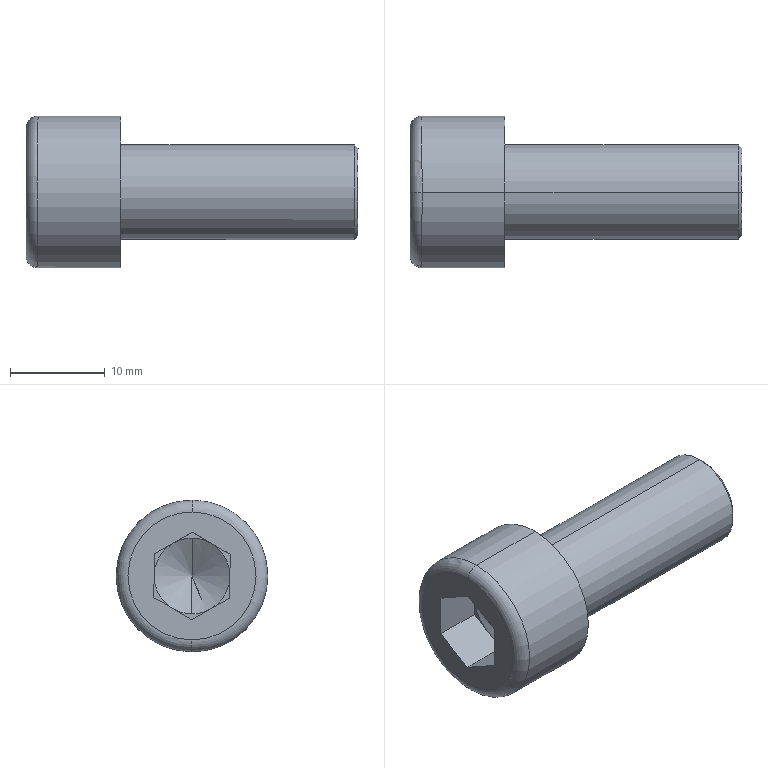Component | SolidWorks | hexagon socket head cap screws gb-29 | 1 solid | 25 faces | box 35.01 x 16 x 16.01 mm | volume 3640 mm3 | plane 15 | cone 4 | cylinder 4 | torus 2 | commonest cylinder face diameters 10 x2 16 x2
STEP:
#1=CARTESIAN_POINT('',(-1.117,35.713,19.655));
#2=VERTEX_POINT('',#1);
#3=CARTESIAN_POINT('',(-1.117,35.71,20.017));
#4=VERTEX_POINT('',#3);
#5=CARTESIAN_POINT('',(-1.117,35.712,19.836));
#6=DIRECTION('',(1.,0.,-0.00108));
#7=DIRECTION('',(-0.00108,0.008644,-1.));
#8=AXIS2_PLACEMENT_3D('',#5,#6,#7);
#9=CIRCLE('',#8,0.1811);
#10=EDGE_CURVE('',#2,#4,#9,.T.);
#11=ORIENTED_EDGE('',*,*,#10,.F.);
#12=CARTESIAN_POINT('',(-1.133,35.714,19.639));
#13=VERTEX_POINT('',#12);
#14=CARTESIAN_POINT('',(-1.117,35.713,19.655));
#15=DIRECTION('',(-0.7079,0.006112,-0.7063));
#16=VECTOR('',#15,39.37);
#17=LINE('',#14,#16);
#18=EDGE_CURVE('',#2,#13,#17,.T.);
#19=ORIENTED_EDGE('',*,*,#18,.T.);
#20=CARTESIAN_POINT('',(-1.133,35.71,20.033));
#21=VERTEX_POINT('',#20);
#22=CARTESIAN_POINT('',(-1.133,35.712,19.836));
#23=DIRECTION('',(-1.,-0.,0.00108));
#24=DIRECTION('',(-0.00108,0.008644,-1.));
#25=AXIS2_PLACEMENT_3D('',#22,#23,#24);
#26=CIRCLE('',#25,0.1969);
#27=EDGE_CURVE('',#21,#13,#26,.T.);
#28=ORIENTED_EDGE('',*,*,#27,.F.);
#29=CARTESIAN_POINT('',(-1.117,35.71,20.017));
#30=DIRECTION('',(-0.7063,-0.006112,0.7078));
#31=VECTOR('',#30,39.37);
#32=LINE('',#29,#31);
#33=EDGE_CURVE('',#4,#21,#32,.T.);
#34=ORIENTED_EDGE('',*,*,#33,.F.);
#35=EDGE_LOOP('',(#11,#19,#28,#34));
#36=FACE_OUTER_BOUND('',#35,.T.);
#37=CARTESIAN_POINT('',(-1.117,35.712,19.836));
#38=DIRECTION('',(-1.,-0.,0.00108));
#39=DIRECTION('',(0.00108,-0.008644,1.));
#40=AXIS2_PLACEMENT_3D('',#37,#38,#39);
#41=CONICAL_SURFACE('',#40,0.1811,0.7854);
#42=ADVANCED_FACE('',(#36),#41,.T.);
#43=CARTESIAN_POINT('',(-2.495,35.71,20.103));
#44=VERTEX_POINT('',#43);
#45=CARTESIAN_POINT('',(-2.495,35.714,19.572));
#46=VERTEX_POINT('',#45);
#47=CARTESIAN_POINT('',(-2.495,35.712,19.837));
#48=DIRECTION('',(-1.,-0.,0.00108));
#49=DIRECTION('',(-0.00108,0.008644,-1.));
#50=AXIS2_PLACEMENT_3D('',#47,#48,#49);
#51=CIRCLE('',#50,0.2657);
#52=EDGE_CURVE('',#44,#46,#51,.T.);
#53=ORIENTED_EDGE('',*,*,#52,.F.);
#54=CARTESIAN_POINT('',(-2.446,35.709,20.152));
#55=VERTEX_POINT('',#54);
#56=CARTESIAN_POINT('',(-2.446,35.71,20.103));
#57=DIRECTION('',(0.00000934,1.,0.008644));
#58=DIRECTION('',(0.,-0.008644,1.));
#59=AXIS2_PLACEMENT_3D('',#56,#57,#58);
#60=CIRCLE('',#59,0.04921);
#61=EDGE_CURVE('',#44,#55,#60,.T.);
#62=ORIENTED_EDGE('',*,*,#61,.T.);
#63=CARTESIAN_POINT('',(-2.446,35.715,19.522));
#64=VERTEX_POINT('',#63);
#65=CARTESIAN_POINT('',(-2.446,35.712,19.837));
#66=DIRECTION('',(1.,0.,-0.00108));
#67=DIRECTION('',(-0.00108,0.008644,-1.));
#68=AXIS2_PLACEMENT_3D('',#65,#66,#67);
#69=CIRCLE('',#68,0.315);
#70=EDGE_CURVE('',#64,#55,#69,.T.);
#71=ORIENTED_EDGE('',*,*,#70,.F.);
#72=CARTESIAN_POINT('',(-2.446,35.714,19.571));
#73=DIRECTION('',(-0.00000934,-1.,-0.008644));
#74=DIRECTION('',(0.,0.008644,-1.));
#75=AXIS2_PLACEMENT_3D('',#72,#73,#74);
#76=CIRCLE('',#75,0.04921);
#77=EDGE_CURVE('',#46,#64,#76,.T.);
#78=ORIENTED_EDGE('',*,*,#77,.F.);
#79=EDGE_LOOP('',(#53,#62,#71,#78));
#80=FACE_OUTER_BOUND('',#79,.T.);
#81=CARTESIAN_POINT('',(-2.446,35.712,19.837));
#82=DIRECTION('',(1.,0.,-0.00108));
#83=DIRECTION('',(-0.00108,0.008644,-1.));
#84=AXIS2_PLACEMENT_3D('',#81,#82,#83);
#85=TOROIDAL_SURFACE('',#84,0.2657,0.04921);
#86=ADVANCED_FACE('',(#80),#85,.T.);
#87=CARTESIAN_POINT('',(-2.207,35.712,19.837));
#88=VERTEX_POINT('',#87);
#89=CARTESIAN_POINT('',(-2.298,35.711,19.994));
#90=VERTEX_POINT('',#89);
#91=CARTESIAN_POINT('',(-2.298,35.711,19.994));
#92=DIRECTION('',(-0.4991,-0.007486,0.8665));
#93=VECTOR('',#92,39.37);
#94=LINE('',#91,#93);
#95=EDGE_CURVE('',#88,#90,#94,.T.);
#96=ORIENTED_EDGE('',*,*,#95,.F.);
#97=CARTESIAN_POINT('',(-2.298,35.713,19.68));
#98=VERTEX_POINT('',#97);
#99=CARTESIAN_POINT('',(-2.298,35.713,19.68));
#100=DIRECTION('',(-0.5009,0.007486,-0.8655));
#101=VECTOR('',#100,39.37);
#102=LINE('',#99,#101);
#103=EDGE_CURVE('',#88,#98,#102,.T.);
#104=ORIENTED_EDGE('',*,*,#103,.T.);
#105=CARTESIAN_POINT('',(-2.298,35.634,19.7));
#106=VERTEX_POINT('',#105);
#107=CARTESIAN_POINT('',(-2.298,35.712,19.837));
#108=DIRECTION('',(1.,0.,-0.00108));
#109=DIRECTION('',(0.00108,-0.008644,1.));
#110=AXIS2_PLACEMENT_3D('',#107,#108,#109);
#111=CIRCLE('',#110,0.1575);
#112=EDGE_CURVE('',#106,#98,#111,.T.);
#113=ORIENTED_EDGE('',*,*,#112,.F.);
#114=CARTESIAN_POINT('',(-2.298,35.554,19.836));
#115=VERTEX_POINT('',#114);
#116=CARTESIAN_POINT('',(-2.298,35.712,19.837));
#117=DIRECTION('',(1.,0.,-0.00108));
#118=DIRECTION('',(0.00108,-0.008644,1.));
#119=AXIS2_PLACEMENT_3D('',#116,#117,#118);
#120=CIRCLE('',#119,0.1575);
#121=EDGE_CURVE('',#115,#106,#120,.T.);
#122=ORIENTED_EDGE('',*,*,#121,.F.);
#123=CARTESIAN_POINT('',(-2.298,35.632,19.973));
#124=VERTEX_POINT('',#123);
#125=CARTESIAN_POINT('',(-2.298,35.712,19.837));
#126=DIRECTION('',(1.,0.,-0.00108));
#127=DIRECTION('',(0.00108,-0.008644,1.));
#128=AXIS2_PLACEMENT_3D('',#125,#126,#127);
#129=CIRCLE('',#128,0.1575);
#130=EDGE_CURVE('',#124,#115,#129,.T.);
#131=ORIENTED_EDGE('',*,*,#130,.F.);
#132=CARTESIAN_POINT('',(-2.298,35.712,19.837));
#133=DIRECTION('',(1.,0.,-0.00108));
#134=DIRECTION('',(0.00108,-0.008644,1.));
#135=AXIS2_PLACEMENT_3D('',#132,#133,#134);
#136=CIRCLE('',#135,0.1575);
#137=EDGE_CURVE('',#90,#124,#136,.T.);
#138=ORIENTED_EDGE('',*,*,#137,.F.);
#139=EDGE_LOOP('',(#96,#104,#113,#122,#131,#138));
#140=FACE_OUTER_BOUND('',#139,.T.);
#141=CARTESIAN_POINT('',(-2.298,35.712,19.837));
#142=DIRECTION('',(-1.,-0.,0.00108));
#143=DIRECTION('',(0.00108,-0.008644,1.));
#144=AXIS2_PLACEMENT_3D('',#141,#142,#143);
#145=CONICAL_SURFACE('',#144,0.1575,1.047);
#146=ADVANCED_FACE('',(#140),#145,.F.);
#147=ORIENTED_EDGE('',*,*,#27,.T.);
#148=CARTESIAN_POINT('',(-2.102,35.714,19.64));
#149=VERTEX_POINT('',#148);
#150=CARTESIAN_POINT('',(-1.117,35.714,19.639));
#151=DIRECTION('',(-1.,-0.,0.00108));
#152=VECTOR('',#151,39.37);
#153=LINE('',#150,#152);
#154=EDGE_CURVE('',#13,#149,#153,.T.);
#155=ORIENTED_EDGE('',*,*,#154,.T.);
#156=CARTESIAN_POINT('',(-2.101,35.71,20.034));
#157=VERTEX_POINT('',#156);
#158=CARTESIAN_POINT('',(-2.101,35.712,19.837));
#159=DIRECTION('',(1.,0.,-0.00108));
#160=DIRECTION('',(-0.00108,0.008644,-1.));
#161=AXIS2_PLACEMENT_3D('',#158,#159,#160);
#162=CIRCLE('',#161,0.1969);
#163=EDGE_CURVE('',#149,#157,#162,.T.);
#164=ORIENTED_EDGE('',*,*,#163,.T.);
#165=CARTESIAN_POINT('',(-1.117,35.71,20.033));
#166=DIRECTION('',(-1.,-0.,0.00108));
#167=VECTOR('',#166,39.37);
#168=LINE('',#165,#167);
#169=EDGE_CURVE('',#21,#157,#168,.T.);
#170=ORIENTED_EDGE('',*,*,#169,.F.);
#171=EDGE_LOOP('',(#147,#155,#164,#170));
#172=FACE_OUTER_BOUND('',#171,.T.);
#173=CARTESIAN_POINT('',(-1.117,35.712,19.836));
#174=DIRECTION('',(-1.,-0.,0.00108));
#175=DIRECTION('',(0.00108,-0.008644,1.));
#176=AXIS2_PLACEMENT_3D('',#173,#174,#175);
#177=CYLINDRICAL_SURFACE('',#176,0.1969);
#178=ADVANCED_FACE('',(#172),#177,.T.);
#179=CARTESIAN_POINT('',(-2.102,35.715,19.522));
#180=VERTEX_POINT('',#179);
#181=CARTESIAN_POINT('',(-2.101,35.709,20.152));
#182=VERTEX_POINT('',#181);
#183=CARTESIAN_POINT('',(-2.101,35.712,19.837));
#184=DIRECTION('',(1.,0.,-0.00108));
#185=DIRECTION('',(-0.00108,0.008644,-1.));
#186=AXIS2_PLACEMENT_3D('',#183,#184,#185);
#187=CIRCLE('',#186,0.315);
#188=EDGE_CURVE('',#180,#182,#187,.T.);
#189=ORIENTED_EDGE('',*,*,#188,.F.);
#190=CARTESIAN_POINT('',(-2.102,35.715,19.522));
#191=DIRECTION('',(-1.,-0.,0.00108));
#192=VECTOR('',#191,39.37);
#193=LINE('',#190,#192);
#194=EDGE_CURVE('',#180,#64,#193,.T.);
#195=ORIENTED_EDGE('',*,*,#194,.T.);
#196=ORIENTED_EDGE('',*,*,#70,.T.);
#197=CARTESIAN_POINT('',(-2.101,35.709,20.152));
#198=DIRECTION('',(-1.,-0.,0.00108));
#199=VECTOR('',#198,39.37);
#200=LINE('',#197,#199);
#201=EDGE_CURVE('',#182,#55,#200,.T.);
#202=ORIENTED_EDGE('',*,*,#201,.F.);
#203=EDGE_LOOP('',(#189,#195,#196,#202));
#204=FACE_OUTER_BOUND('',#203,.T.);
#205=CARTESIAN_POINT('',(-2.101,35.712,19.837));
#206=DIRECTION('',(-1.,-0.,0.00108));
#207=DIRECTION('',(0.00108,-0.008644,1.));
#208=AXIS2_PLACEMENT_3D('',#205,#206,#207);
#209=CYLINDRICAL_SURFACE('',#208,0.315);
#210=ADVANCED_FACE('',(#204),#209,.T.);
#211=CARTESIAN_POINT('',(-2.298,35.554,19.927));
#212=VERTEX_POINT('',#211);
#213=CARTESIAN_POINT('',(-2.298,35.71,20.019));
#214=DIRECTION('',(-0.0005483,-0.8617,-0.5075));
#215=VECTOR('',#214,39.37);
#216=LINE('',#213,#215);
#217=EDGE_CURVE('',#124,#212,#216,.T.);
#218=ORIENTED_EDGE('',*,*,#217,.F.);
#219=ORIENTED_EDGE('',*,*,#130,.T.);
#220=CARTESIAN_POINT('',(-2.298,35.554,19.927));
#221=DIRECTION('',(-0.00108,0.008644,-1.));
#222=VECTOR('',#221,39.37);
#223=LINE('',#220,#222);
#224=EDGE_CURVE('',#212,#115,#223,.T.);
#225=ORIENTED_EDGE('',*,*,#224,.F.);
#226=EDGE_LOOP('',(#218,#219,#225));
#227=FACE_OUTER_BOUND('',#226,.T.);
#228=CARTESIAN_POINT('',(-2.298,35.397,19.834));
#229=DIRECTION('',(-1.,-0.,0.00108));
#230=DIRECTION('',(0.00108,-0.008644,1.));
#231=AXIS2_PLACEMENT_3D('',#228,#229,#230);
#232=PLANE('',#231);
#233=ADVANCED_FACE('',(#227),#232,.T.);
#234=CARTESIAN_POINT('',(-2.298,35.555,19.745));
#235=VERTEX_POINT('',#234);
#236=CARTESIAN_POINT('',(-2.298,35.554,19.927));
#237=DIRECTION('',(-0.00108,0.008644,-1.));
#238=VECTOR('',#237,39.37);
#239=LINE('',#236,#238);
#240=EDGE_CURVE('',#115,#235,#239,.T.);
#241=ORIENTED_EDGE('',*,*,#240,.F.);
#242=ORIENTED_EDGE('',*,*,#121,.T.);
#243=CARTESIAN_POINT('',(-2.298,35.555,19.745));
#244=DIRECTION('',(-0.0005321,0.8703,-0.4925));
#245=VECTOR('',#244,39.37);
#246=LINE('',#243,#245);
#247=EDGE_CURVE('',#235,#106,#246,.T.);
#248=ORIENTED_EDGE('',*,*,#247,.F.);
#249=EDGE_LOOP('',(#241,#242,#248));
#250=FACE_OUTER_BOUND('',#249,.T.);
#251=CARTESIAN_POINT('',(-2.298,35.397,19.834));
#252=DIRECTION('',(-1.,-0.,0.00108));
#253=DIRECTION('',(0.00108,-0.008644,1.));
#254=AXIS2_PLACEMENT_3D('',#251,#252,#253);
#255=PLANE('',#254);
#256=ADVANCED_FACE('',(#250),#255,.T.);
#257=CARTESIAN_POINT('',(-2.298,35.713,19.655));
#258=VERTEX_POINT('',#257);
#259=CARTESIAN_POINT('',(-2.298,35.555,19.745));
#260=DIRECTION('',(-0.0005321,0.8703,-0.4925));
#261=VECTOR('',#260,39.37);
#262=LINE('',#259,#261);
#263=EDGE_CURVE('',#106,#258,#262,.T.);
#264=ORIENTED_EDGE('',*,*,#263,.F.);
#265=ORIENTED_EDGE('',*,*,#112,.T.);
#266=CARTESIAN_POINT('',(-2.298,35.792,19.701));
#267=VERTEX_POINT('',#266);
#268=CARTESIAN_POINT('',(-2.298,35.712,19.837));
#269=DIRECTION('',(1.,0.,-0.00108));
#270=DIRECTION('',(0.00108,-0.008644,1.));
#271=AXIS2_PLACEMENT_3D('',#268,#269,#270);
#272=CIRCLE('',#271,0.1575);
#273=EDGE_CURVE('',#98,#267,#272,.T.);
#274=ORIENTED_EDGE('',*,*,#273,.T.);
#275=CARTESIAN_POINT('',(-2.298,35.713,19.655));
#276=DIRECTION('',(0.0005483,0.8617,0.5075));
#277=VECTOR('',#276,39.37);
#278=LINE('',#275,#277);
#279=EDGE_CURVE('',#258,#267,#278,.T.);
#280=ORIENTED_EDGE('',*,*,#279,.F.);
#281=EDGE_LOOP('',(#264,#265,#274,#280));
#282=FACE_OUTER_BOUND('',#281,.T.);
#283=CARTESIAN_POINT('',(-2.298,35.397,19.834));
#284=DIRECTION('',(-1.,-0.,0.00108));
#285=DIRECTION('',(0.00108,-0.008644,1.));
#286=AXIS2_PLACEMENT_3D('',#283,#284,#285);
#287=PLANE('',#286);
#288=ADVANCED_FACE('',(#282),#287,.T.);
#289=CARTESIAN_POINT('',(-2.298,35.87,19.747));
#290=VERTEX_POINT('',#289);
#291=CARTESIAN_POINT('',(-2.298,35.713,19.655));
#292=DIRECTION('',(0.0005483,0.8617,0.5075));
#293=VECTOR('',#292,39.37);
#294=LINE('',#291,#293);
#295=EDGE_CURVE('',#267,#290,#294,.T.);
#296=ORIENTED_EDGE('',*,*,#295,.F.);
#297=CARTESIAN_POINT('',(-2.298,35.869,19.838));
#298=VERTEX_POINT('',#297);
#299=CARTESIAN_POINT('',(-2.298,35.712,19.837));
#300=DIRECTION('',(1.,0.,-0.00108));
#301=DIRECTION('',(-0.00108,0.008644,-1.));
#302=AXIS2_PLACEMENT_3D('',#299,#300,#301);
#303=CIRCLE('',#302,0.1575);
#304=EDGE_CURVE('',#267,#298,#303,.T.);
#305=ORIENTED_EDGE('',*,*,#304,.T.);
#306=CARTESIAN_POINT('',(-2.298,35.87,19.747));
#307=DIRECTION('',(0.00108,-0.008644,1.));
#308=VECTOR('',#307,39.37);
#309=LINE('',#306,#308);
#310=EDGE_CURVE('',#290,#298,#309,.T.);
#311=ORIENTED_EDGE('',*,*,#310,.F.);
#312=EDGE_LOOP('',(#296,#305,#311));
#313=FACE_OUTER_BOUND('',#312,.T.);
#314=CARTESIAN_POINT('',(-2.298,35.397,19.834));
#315=DIRECTION('',(-1.,-0.,0.00108));
#316=DIRECTION('',(0.00108,-0.008644,1.));
#317=AXIS2_PLACEMENT_3D('',#314,#315,#316);
#318=PLANE('',#317);
#319=ADVANCED_FACE('',(#313),#318,.T.);
#320=CARTESIAN_POINT('',(-2.298,35.869,19.929));
#321=VERTEX_POINT('',#320);
#322=CARTESIAN_POINT('',(-2.298,35.87,19.747));
#323=DIRECTION('',(0.00108,-0.008644,1.));
#324=VECTOR('',#323,39.37);
#325=LINE('',#322,#324);
#326=EDGE_CURVE('',#298,#321,#325,.T.);
#327=ORIENTED_EDGE('',*,*,#326,.F.);
#328=CARTESIAN_POINT('',(-2.298,35.789,19.974));
#329=VERTEX_POINT('',#328);
#330=CARTESIAN_POINT('',(-2.298,35.712,19.837));
#331=DIRECTION('',(1.,0.,-0.00108));
#332=DIRECTION('',(0.00108,-0.008644,1.));
#333=AXIS2_PLACEMENT_3D('',#330,#331,#332);
#334=CIRCLE('',#333,0.1575);
#335=EDGE_CURVE('',#298,#329,#334,.T.);
#336=ORIENTED_EDGE('',*,*,#335,.T.);
#337=CARTESIAN_POINT('',(-2.298,35.869,19.929));
#338=DIRECTION('',(0.0005321,-0.8703,0.4925));
#339=VECTOR('',#338,39.37);
#340=LINE('',#337,#339);
#341=EDGE_CURVE('',#321,#329,#340,.T.);
#342=ORIENTED_EDGE('',*,*,#341,.F.);
#343=EDGE_LOOP('',(#327,#336,#342));
#344=FACE_OUTER_BOUND('',#343,.T.);
#345=CARTESIAN_POINT('',(-2.298,35.397,19.834));
#346=DIRECTION('',(-1.,-0.,0.00108));
#347=DIRECTION('',(0.00108,-0.008644,1.));
#348=AXIS2_PLACEMENT_3D('',#345,#346,#347);
#349=PLANE('',#348);
#350=ADVANCED_FACE('',(#344),#349,.T.);
#351=CARTESIAN_POINT('',(-2.298,35.71,20.019));
#352=VERTEX_POINT('',#351);
#353=CARTESIAN_POINT('',(-2.298,35.869,19.929));
#354=DIRECTION('',(0.0005321,-0.8703,0.4925));
#355=VECTOR('',#354,39.37);
#356=LINE('',#353,#355);
#357=EDGE_CURVE('',#329,#352,#356,.T.);
#358=ORIENTED_EDGE('',*,*,#357,.F.);
#359=CARTESIAN_POINT('',(-2.298,35.712,19.837));
#360=DIRECTION('',(1.,0.,-0.00108));
#361=DIRECTION('',(0.00108,-0.008644,1.));
#362=AXIS2_PLACEMENT_3D('',#359,#360,#361);
#363=CIRCLE('',#362,0.1575);
#364=EDGE_CURVE('',#329,#90,#363,.T.);
#365=ORIENTED_EDGE('',*,*,#364,.T.);
#366=ORIENTED_EDGE('',*,*,#137,.T.);
#367=CARTESIAN_POINT('',(-2.298,35.71,20.019));
#368=DIRECTION('',(-0.0005483,-0.8617,-0.5075));
#369=VECTOR('',#368,39.37);
#370=LINE('',#367,#369);
#371=EDGE_CURVE('',#352,#124,#370,.T.);
#372=ORIENTED_EDGE('',*,*,#371,.F.);
#373=EDGE_LOOP('',(#358,#365,#366,#372));
#374=FACE_OUTER_BOUND('',#373,.T.);
#375=CARTESIAN_POINT('',(-2.298,35.397,19.834));
#376=DIRECTION('',(-1.,-0.,0.00108));
#377=DIRECTION('',(0.00108,-0.008644,1.));
#378=AXIS2_PLACEMENT_3D('',#375,#376,#377);
#379=PLANE('',#378);
#380=ADVANCED_FACE('',(#374),#379,.T.);
#381=CARTESIAN_POINT('',(-2.495,35.712,19.837));
#382=DIRECTION('',(-1.,-0.,0.00108));
#383=DIRECTION('',(-0.00108,0.008644,-1.));
#384=AXIS2_PLACEMENT_3D('',#381,#382,#383);
#385=CIRCLE('',#384,0.2657);
#386=EDGE_CURVE('',#46,#44,#385,.T.);
#387=ORIENTED_EDGE('',*,*,#386,.T.);
#388=ORIENTED_EDGE('',*,*,#52,.T.);
#389=EDGE_LOOP('',(#387,#388));
#390=FACE_OUTER_BOUND('',#389,.T.);
#391=CARTESIAN_POINT('',(-2.495,35.555,19.745));
#392=VERTEX_POINT('',#391);
#393=CARTESIAN_POINT('',(-2.495,35.713,19.655));
#394=VERTEX_POINT('',#393);
#395=CARTESIAN_POINT('',(-2.495,35.555,19.745));
#396=DIRECTION('',(-0.0005321,0.8703,-0.4925));
#397=VECTOR('',#396,39.37);
#398=LINE('',#395,#397);
#399=EDGE_CURVE('',#392,#394,#398,.T.);
#400=ORIENTED_EDGE('',*,*,#399,.T.);
#401=CARTESIAN_POINT('',(-2.495,35.87,19.748));
#402=VERTEX_POINT('',#401);
#403=CARTESIAN_POINT('',(-2.495,35.713,19.655));
#404=DIRECTION('',(0.0005483,0.8617,0.5075));
#405=VECTOR('',#404,39.37);
#406=LINE('',#403,#405);
#407=EDGE_CURVE('',#394,#402,#406,.T.);
#408=ORIENTED_EDGE('',*,*,#407,.T.);
#409=CARTESIAN_POINT('',(-2.495,35.869,19.93));
#410=VERTEX_POINT('',#409);
#411=CARTESIAN_POINT('',(-2.495,35.87,19.748));
#412=DIRECTION('',(0.00108,-0.008644,1.));
#413=VECTOR('',#412,39.37);
#414=LINE('',#411,#413);
#415=EDGE_CURVE('',#402,#410,#414,.T.);
#416=ORIENTED_EDGE('',*,*,#415,.T.);
#417=CARTESIAN_POINT('',(-2.495,35.71,20.019));
#418=VERTEX_POINT('',#417);
#419=CARTESIAN_POINT('',(-2.495,35.869,19.93));
#420=DIRECTION('',(0.0005321,-0.8703,0.4925));
#421=VECTOR('',#420,39.37);
#422=LINE('',#419,#421);
#423=EDGE_CURVE('',#410,#418,#422,.T.);
#424=ORIENTED_EDGE('',*,*,#423,.T.);
#425=CARTESIAN_POINT('',(-2.495,35.554,19.927));
#426=VERTEX_POINT('',#425);
#427=CARTESIAN_POINT('',(-2.495,35.71,20.019));
#428=DIRECTION('',(-0.0005483,-0.8617,-0.5075));
#429=VECTOR('',#428,39.37);
#430=LINE('',#427,#429);
#431=EDGE_CURVE('',#418,#426,#430,.T.);
#432=ORIENTED_EDGE('',*,*,#431,.T.);
#433=CARTESIAN_POINT('',(-2.495,35.554,19.927));
#434=DIRECTION('',(-0.00108,0.008644,-1.));
#435=VECTOR('',#434,39.37);
#436=LINE('',#433,#435);
#437=EDGE_CURVE('',#426,#392,#436,.T.);
#438=ORIENTED_EDGE('',*,*,#437,.T.);
#439=EDGE_LOOP('',(#400,#408,#416,#424,#432,#438));
#440=FACE_BOUND('',#439,.T.);
#441=CARTESIAN_POINT('',(-2.495,35.712,19.837));
#442=DIRECTION('',(1.,0.,-0.00108));
#443=DIRECTION('',(-0.00108,0.008644,-1.));
#444=AXIS2_PLACEMENT_3D('',#441,#442,#443);
#445=PLANE('',#444);
#446=ADVANCED_FACE('',(#390,#440),#445,.F.);
#447=CARTESIAN_POINT('',(-2.101,35.712,19.837));
#448=DIRECTION('',(1.,0.,-0.00108));
#449=DIRECTION('',(-0.00108,0.008644,-1.));
#450=AXIS2_PLACEMENT_3D('',#447,#448,#449);
#451=CIRCLE('',#450,0.315);
#452=EDGE_CURVE('',#182,#180,#451,.T.);
#453=ORIENTED_EDGE('',*,*,#452,.T.);
#454=ORIENTED_EDGE('',*,*,#188,.T.);
#455=EDGE_LOOP('',(#453,#454));
#456=FACE_OUTER_BOUND('',#455,.T.);
#457=CARTESIAN_POINT('',(-2.101,35.712,19.837));
#458=DIRECTION('',(1.,0.,-0.00108));
#459=DIRECTION('',(-0.00108,0.008644,-1.));
#460=AXIS2_PLACEMENT_3D('',#457,#458,#459);
#461=CIRCLE('',#460,0.1969);
#462=EDGE_CURVE('',#157,#149,#461,.T.);
#463=ORIENTED_EDGE('',*,*,#462,.F.);
#464=ORIENTED_EDGE('',*,*,#163,.F.);
#465=EDGE_LOOP('',(#463,#464));
#466=FACE_BOUND('',#465,.T.);
#467=CARTESIAN_POINT('',(-2.101,35.712,19.837));
#468=DIRECTION('',(1.,0.,-0.00108));
#469=DIRECTION('',(-0.00108,0.008644,-1.));
#470=AXIS2_PLACEMENT_3D('',#467,#468,#469);
#471=PLANE('',#470);
#472=ADVANCED_FACE('',(#456,#466),#471,.T.);
#473=ORIENTED_EDGE('',*,*,#194,.F.);
#474=ORIENTED_EDGE('',*,*,#452,.F.);
#475=ORIENTED_EDGE('',*,*,#201,.T.);
#476=CARTESIAN_POINT('',(-2.446,35.712,19.837));
#477=DIRECTION('',(1.,0.,-0.00108));
#478=DIRECTION('',(-0.00108,0.008644,-1.));
#479=AXIS2_PLACEMENT_3D('',#476,#477,#478);
#480=CIRCLE('',#479,0.315);
#481=EDGE_CURVE('',#55,#64,#480,.T.);
#482=ORIENTED_EDGE('',*,*,#481,.T.);
#483=EDGE_LOOP('',(#473,#474,#475,#482));
#484=FACE_OUTER_BOUND('',#483,.T.);
#485=CARTESIAN_POINT('',(-2.101,35.712,19.837));
#486=DIRECTION('',(-1.,-0.,0.00108));
#487=DIRECTION('',(0.00108,-0.008644,1.));
#488=AXIS2_PLACEMENT_3D('',#485,#486,#487);
#489=CYLINDRICAL_SURFACE('',#488,0.315);
#490=ADVANCED_FACE('',(#484),#489,.T.);
#491=ORIENTED_EDGE('',*,*,#154,.F.);
#492=CARTESIAN_POINT('',(-1.133,35.712,19.836));
#493=DIRECTION('',(-1.,-0.,0.00108));
#494=DIRECTION('',(-0.00108,0.008644,-1.));
#495=AXIS2_PLACEMENT_3D('',#492,#493,#494);
#496=CIRCLE('',#495,0.1969);
#497=EDGE_CURVE('',#13,#21,#496,.T.);
#498=ORIENTED_EDGE('',*,*,#497,.T.);
#499=ORIENTED_EDGE('',*,*,#169,.T.);
#500=ORIENTED_EDGE('',*,*,#462,.T.);
#501=EDGE_LOOP('',(#491,#498,#499,#500));
#502=FACE_OUTER_BOUND('',#501,.T.);
#503=CARTESIAN_POINT('',(-1.117,35.712,19.836));
#504=DIRECTION('',(-1.,-0.,0.00108));
#505=DIRECTION('',(0.00108,-0.008644,1.));
#506=AXIS2_PLACEMENT_3D('',#503,#504,#505);
#507=CYLINDRICAL_SURFACE('',#506,0.1969);
#508=ADVANCED_FACE('',(#502),#507,.T.);
#509=CARTESIAN_POINT('',(-1.117,35.712,19.836));
#510=DIRECTION('',(1.,0.,-0.00108));
#511=DIRECTION('',(-0.00108,0.008644,-1.));
#512=AXIS2_PLACEMENT_3D('',#509,#510,#511);
#513=CIRCLE('',#512,0.1811);
#514=EDGE_CURVE('',#4,#2,#513,.T.);
#515=ORIENTED_EDGE('',*,*,#514,.T.);
#516=ORIENTED_EDGE('',*,*,#10,.T.);
#517=EDGE_LOOP('',(#515,#516));
#518=FACE_OUTER_BOUND('',#517,.T.);
#519=CARTESIAN_POINT('',(-1.117,35.712,19.836));
#520=DIRECTION('',(1.,0.,-0.00108));
#521=DIRECTION('',(-0.00108,0.008644,-1.));
#522=AXIS2_PLACEMENT_3D('',#519,#520,#521);
#523=PLANE('',#522);
#524=ADVANCED_FACE('',(#518),#523,.T.);
#525=ORIENTED_EDGE('',*,*,#399,.F.);
#526=CARTESIAN_POINT('',(-2.298,35.555,19.745));
#527=DIRECTION('',(-1.,-0.,0.00108));
#528=VECTOR('',#527,39.37);
#529=LINE('',#526,#528);
#530=EDGE_CURVE('',#235,#392,#529,.T.);
#531=ORIENTED_EDGE('',*,*,#530,.F.);
#532=ORIENTED_EDGE('',*,*,#247,.T.);
#533=ORIENTED_EDGE('',*,*,#263,.T.);
#534=CARTESIAN_POINT('',(-2.298,35.713,19.655));
#535=DIRECTION('',(-1.,-0.,0.00108));
#536=VECTOR('',#535,39.37);
#537=LINE('',#534,#536);
#538=EDGE_CURVE('',#258,#394,#537,.T.);
#539=ORIENTED_EDGE('',*,*,#538,.T.);
#540=EDGE_LOOP('',(#525,#531,#532,#533,#539));
#541=FACE_OUTER_BOUND('',#540,.T.);
#542=CARTESIAN_POINT('',(-2.298,35.555,19.745));
#543=DIRECTION('',(0.0009403,0.4925,0.8703));
#544=DIRECTION('',(0.0005321,-0.8703,0.4925));
#545=AXIS2_PLACEMENT_3D('',#542,#543,#544);
#546=PLANE('',#545);
#547=ADVANCED_FACE('',(#541),#546,.T.);
#548=ORIENTED_EDGE('',*,*,#407,.F.);
#549=ORIENTED_EDGE('',*,*,#538,.F.);
#550=ORIENTED_EDGE('',*,*,#279,.T.);
#551=ORIENTED_EDGE('',*,*,#295,.T.);
#552=CARTESIAN_POINT('',(-2.298,35.87,19.747));
#553=DIRECTION('',(-1.,-0.,0.00108));
#554=VECTOR('',#553,39.37);
#555=LINE('',#552,#554);
#556=EDGE_CURVE('',#290,#402,#555,.T.);
#557=ORIENTED_EDGE('',*,*,#556,.T.);
#558=EDGE_LOOP('',(#548,#549,#550,#551,#557));
#559=FACE_OUTER_BOUND('',#558,.T.);
#560=CARTESIAN_POINT('',(-2.298,35.713,19.655));
#561=DIRECTION('',(0.000931,-0.5075,0.8617));
#562=DIRECTION('',(-0.0005483,-0.8617,-0.5075));
#563=AXIS2_PLACEMENT_3D('',#560,#561,#562);
#564=PLANE('',#563);
#565=ADVANCED_FACE('',(#559),#564,.T.);
#566=ORIENTED_EDGE('',*,*,#415,.F.);
#567=ORIENTED_EDGE('',*,*,#556,.F.);
#568=ORIENTED_EDGE('',*,*,#310,.T.);
#569=ORIENTED_EDGE('',*,*,#326,.T.);
#570=CARTESIAN_POINT('',(-2.298,35.869,19.929));
#571=DIRECTION('',(-1.,-0.,0.00108));
#572=VECTOR('',#571,39.37);
#573=LINE('',#570,#572);
#574=EDGE_CURVE('',#321,#410,#573,.T.);
#575=ORIENTED_EDGE('',*,*,#574,.T.);
#576=EDGE_LOOP('',(#566,#567,#568,#569,#575));
#577=FACE_OUTER_BOUND('',#576,.T.);
#578=CARTESIAN_POINT('',(-2.298,35.87,19.747));
#579=DIRECTION('',(-0.00000934,-1.,-0.008644));
#580=DIRECTION('',(-0.00108,0.008644,-1.));
#581=AXIS2_PLACEMENT_3D('',#578,#579,#580);
#582=PLANE('',#581);
#583=ADVANCED_FACE('',(#577),#582,.T.);
#584=ORIENTED_EDGE('',*,*,#423,.F.);
#585=ORIENTED_EDGE('',*,*,#574,.F.);
#586=ORIENTED_EDGE('',*,*,#341,.T.);
#587=ORIENTED_EDGE('',*,*,#357,.T.);
#588=CARTESIAN_POINT('',(-2.298,35.71,20.019));
#589=DIRECTION('',(-1.,-0.,0.00108));
#590=VECTOR('',#589,39.37);
#591=LINE('',#588,#590);
#592=EDGE_CURVE('',#352,#418,#591,.T.);
#593=ORIENTED_EDGE('',*,*,#592,.T.);
#594=EDGE_LOOP('',(#584,#585,#586,#587,#593));
#595=FACE_OUTER_BOUND('',#594,.T.);
#596=CARTESIAN_POINT('',(-2.298,35.869,19.929));
#597=DIRECTION('',(-0.0009403,-0.4925,-0.8703));
#598=DIRECTION('',(-0.0005321,0.8703,-0.4925));
#599=AXIS2_PLACEMENT_3D('',#596,#597,#598);
#600=PLANE('',#599);
#601=ADVANCED_FACE('',(#595),#600,.T.);
#602=ORIENTED_EDGE('',*,*,#431,.F.);
#603=ORIENTED_EDGE('',*,*,#592,.F.);
#604=ORIENTED_EDGE('',*,*,#371,.T.);
#605=ORIENTED_EDGE('',*,*,#217,.T.);
#606=CARTESIAN_POINT('',(-2.298,35.554,19.927));
#607=DIRECTION('',(-1.,-0.,0.00108));
#608=VECTOR('',#607,39.37);
#609=LINE('',#606,#608);
#610=EDGE_CURVE('',#212,#426,#609,.T.);
#611=ORIENTED_EDGE('',*,*,#610,.T.);
#612=EDGE_LOOP('',(#602,#603,#604,#605,#611));
#613=FACE_OUTER_BOUND('',#612,.T.);
#614=CARTESIAN_POINT('',(-2.298,35.71,20.019));
#615=DIRECTION('',(-0.000931,0.5075,-0.8617));
#616=DIRECTION('',(0.0005483,0.8617,0.5075));
#617=AXIS2_PLACEMENT_3D('',#614,#615,#616);
#618=PLANE('',#617);
#619=ADVANCED_FACE('',(#613),#618,.T.);
#620=ORIENTED_EDGE('',*,*,#437,.F.);
#621=ORIENTED_EDGE('',*,*,#610,.F.);
#622=ORIENTED_EDGE('',*,*,#224,.T.);
#623=ORIENTED_EDGE('',*,*,#240,.T.);
#624=ORIENTED_EDGE('',*,*,#530,.T.);
#625=EDGE_LOOP('',(#620,#621,#622,#623,#624));
#626=FACE_OUTER_BOUND('',#625,.T.);
#627=CARTESIAN_POINT('',(-2.298,35.554,19.927));
#628=DIRECTION('',(0.00000934,1.,0.008644));
#629=DIRECTION('',(0.00108,-0.008644,1.));
#630=AXIS2_PLACEMENT_3D('',#627,#628,#629);
#631=PLANE('',#630);
#632=ADVANCED_FACE('',(#626),#631,.T.);
#633=ORIENTED_EDGE('',*,*,#103,.F.);
#634=ORIENTED_EDGE('',*,*,#95,.T.);
#635=ORIENTED_EDGE('',*,*,#364,.F.);
#636=ORIENTED_EDGE('',*,*,#335,.F.);
#637=ORIENTED_EDGE('',*,*,#304,.F.);
#638=ORIENTED_EDGE('',*,*,#273,.F.);
#639=EDGE_LOOP('',(#633,#634,#635,#636,#637,#638));
#640=FACE_OUTER_BOUND('',#639,.T.);
#641=CARTESIAN_POINT('',(-2.298,35.712,19.837));
#642=DIRECTION('',(-1.,-0.,0.00108));
#643=DIRECTION('',(0.00108,-0.008644,1.));
#644=AXIS2_PLACEMENT_3D('',#641,#642,#643);
#645=CONICAL_SURFACE('',#644,0.1575,1.047);
#646=ADVANCED_FACE('',(#640),#645,.F.);
#647=ORIENTED_EDGE('',*,*,#61,.F.);
#648=ORIENTED_EDGE('',*,*,#386,.F.);
#649=ORIENTED_EDGE('',*,*,#77,.T.);
#650=ORIENTED_EDGE('',*,*,#481,.F.);
#651=EDGE_LOOP('',(#647,#648,#649,#650));
#652=FACE_OUTER_BOUND('',#651,.T.);
#653=CARTESIAN_POINT('',(-2.446,35.712,19.837));
#654=DIRECTION('',(1.,0.,-0.00108));
#655=DIRECTION('',(-0.00108,0.008644,-1.));
#656=AXIS2_PLACEMENT_3D('',#653,#654,#655);
#657=TOROIDAL_SURFACE('',#656,0.2657,0.04921);
#658=ADVANCED_FACE('',(#652),#657,.T.);
#659=ORIENTED_EDGE('',*,*,#18,.F.);
#660=ORIENTED_EDGE('',*,*,#514,.F.);
#661=ORIENTED_EDGE('',*,*,#33,.T.);
#662=ORIENTED_EDGE('',*,*,#497,.F.);
#663=EDGE_LOOP('',(#659,#660,#661,#662));
#664=FACE_OUTER_BOUND('',#663,.T.);
#665=CARTESIAN_POINT('',(-1.117,35.712,19.836));
#666=DIRECTION('',(-1.,-0.,0.00108));
#667=DIRECTION('',(0.00108,-0.008644,1.));
#668=AXIS2_PLACEMENT_3D('',#665,#666,#667);
#669=CONICAL_SURFACE('',#668,0.1811,0.7854);
#670=ADVANCED_FACE('',(#664),#669,.T.);
#671=CLOSED_SHELL('',(#42,#86,#146,#178,#210,#233,#256,#288,#319,#350,#380,#446,#472,#490,#508,#524,#547,#565,#583,#601,#619,#632,#646,#658,#670));
#672=MANIFOLD_SOLID_BREP('',#671);
#673=CARTESIAN_POINT('',(0.,0.,0.));
#674=DIRECTION('',(0.,0.,1.));
#675=DIRECTION('',(1.,0.,0.));
#676=AXIS2_PLACEMENT_3D('',#673,#674,#675);
#677=(LENGTH_UNIT()NAMED_UNIT(*)SI_UNIT($,.METRE.));
#678=LENGTH_MEASURE_WITH_UNIT(LENGTH_MEASURE(0.0254),#677);
#679=DIMENSIONAL_EXPONENTS(1.,0.,0.,0.,0.,0.,0.);
#680=(CONVERSION_BASED_UNIT('',#678)LENGTH_UNIT()NAMED_UNIT(#679));
#681=UNCERTAINTY_MEASURE_WITH_UNIT(LENGTH_MEASURE(0.00001),#680,'','');
#682=(NAMED_UNIT(*)PLANE_ANGLE_UNIT()SI_UNIT($,.RADIAN.));
#683=(NAMED_UNIT(*)SI_UNIT($,.STERADIAN.)SOLID_ANGLE_UNIT());
#684=(GEOMETRIC_REPRESENTATION_CONTEXT(3)GLOBAL_UNCERTAINTY_ASSIGNED_CONTEXT((#681))GLOBAL_UNIT_ASSIGNED_CONTEXT((#680,#682,#683))REPRESENTATION_CONTEXT('',''));
#685=ADVANCED_BREP_SHAPE_REPRESENTATION('',(#672,#676),#684);
#686=COLOUR_RGB('',0.7922,0.8196,0.9333);
#687=FILL_AREA_STYLE_COLOUR('',#686);
#688=FILL_AREA_STYLE('',(#687));
#689=SURFACE_STYLE_FILL_AREA(#688);
#690=SURFACE_SIDE_STYLE('',(#689));
#691=SURFACE_STYLE_USAGE(.BOTH.,#690);
#692=PRESENTATION_STYLE_ASSIGNMENT((#691));
#693=STYLED_ITEM('',(#692),#672);
#694=PRESENTATION_LAYER_ASSIGNMENT('','',(#693));
#695=(LENGTH_UNIT()NAMED_UNIT(*)SI_UNIT($,.METRE.));
#696=LENGTH_MEASURE_WITH_UNIT(LENGTH_MEASURE(0.0254),#695);
#697=DIMENSIONAL_EXPONENTS(1.,0.,0.,0.,0.,0.,0.);
#698=(CONVERSION_BASED_UNIT('',#696)LENGTH_UNIT()NAMED_UNIT(#697));
#699=UNCERTAINTY_MEASURE_WITH_UNIT(LENGTH_MEASURE(0.00001),#698,'','');
#700=(NAMED_UNIT(*)PLANE_ANGLE_UNIT()SI_UNIT($,.RADIAN.));
#701=(NAMED_UNIT(*)SI_UNIT($,.STERADIAN.)SOLID_ANGLE_UNIT());
#702=(GEOMETRIC_REPRESENTATION_CONTEXT(3)GLOBAL_UNCERTAINTY_ASSIGNED_CONTEXT((#699))GLOBAL_UNIT_ASSIGNED_CONTEXT((#698,#700,#701))REPRESENTATION_CONTEXT('',''));
#703=MECHANICAL_DESIGN_GEOMETRIC_PRESENTATION_REPRESENTATION('',(#693),#702);